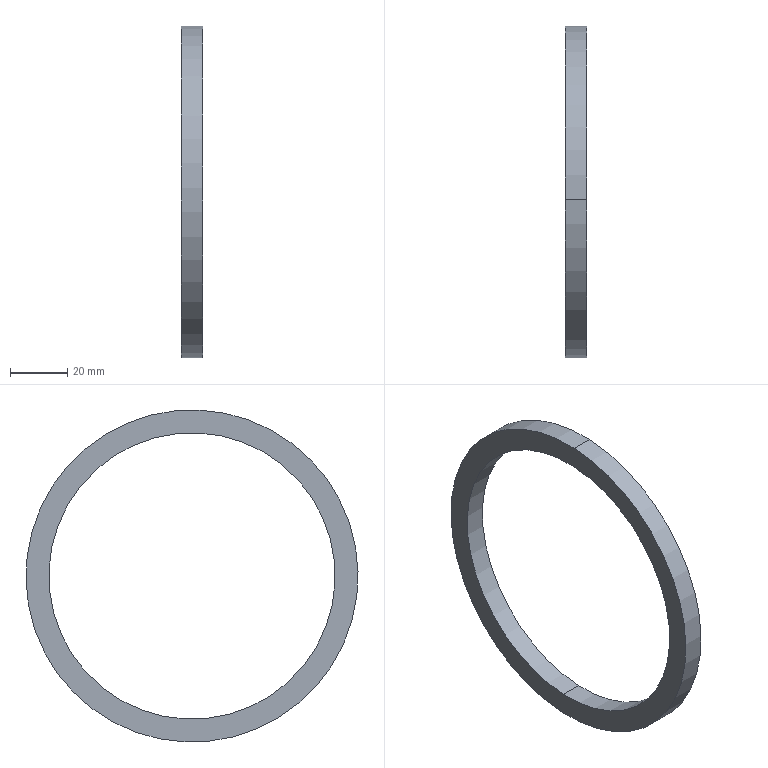Component | SolidWorks | SealRing1-1 | 1 solid | 6 faces | box 7.5 x 116 x 116 mm | volume 20358 mm3 | cylinder 4 | plane 2 | commonest cylinder face diameters 100 x2 116 x2
build123d program:
from build123d import *

# Parameters (mm, degrees)
SKETCH2_R           = 58
SKETCH2_R_2         = 50
BOSS_EXTRUDE1_DEPTH = 7.5


with BuildPart() as part:
    # Sketch2 → Boss-Extrude1 (new body)
    with BuildSketch(Plane(origin=(0, 0, 0), x_dir=(0, 0, -1), z_dir=(1, 0, 0))):
        Circle(SKETCH2_R)
        Circle(SKETCH2_R_2, mode=Mode.SUBTRACT)
    extrude(amount=BOSS_EXTRUDE1_DEPTH)


solid = part.part

# Placed as in the assembly
solid = solid.moved(Location((-138, 0, 0), (0, 0, 0)))
STEP:
#1=COLOUR_RGB('',0.7922,0.8196,0.9333);
#2=FILL_AREA_STYLE_COLOUR('',#1);
#3=FILL_AREA_STYLE('',(#2));
#4=SURFACE_STYLE_FILL_AREA(#3);
#5=SURFACE_SIDE_STYLE('',(#4));
#6=SURFACE_STYLE_USAGE(.BOTH.,#5);
#7=PRESENTATION_STYLE_ASSIGNMENT((#6));
#8=CARTESIAN_POINT('',(-5.138,-0.09506,1.966));
#9=VERTEX_POINT('',#8);
#10=CARTESIAN_POINT('',(-5.138,0.09506,-1.966));
#11=VERTEX_POINT('',#10);
#12=CARTESIAN_POINT('',(-5.138,-0.,0.));
#13=DIRECTION('',(1.,0.,-0.));
#14=DIRECTION('',(-0.,0.04829,-0.9988));
#15=AXIS2_PLACEMENT_3D('',#12,#13,#14);
#16=CIRCLE('',#15,1.969);
#17=EDGE_CURVE('',#9,#11,#16,.T.);
#18=ORIENTED_EDGE('',*,*,#17,.T.);
#19=CARTESIAN_POINT('',(-5.433,0.09506,-1.966));
#20=VERTEX_POINT('',#19);
#21=CARTESIAN_POINT('',(-5.138,0.09506,-1.966));
#22=DIRECTION('',(-1.,-0.,0.));
#23=VECTOR('',#22,39.37);
#24=LINE('',#21,#23);
#25=EDGE_CURVE('',#11,#20,#24,.T.);
#26=ORIENTED_EDGE('',*,*,#25,.T.);
#27=CARTESIAN_POINT('',(-5.433,-0.09506,1.966));
#28=VERTEX_POINT('',#27);
#29=CARTESIAN_POINT('',(-5.433,-0.,0.));
#30=DIRECTION('',(1.,0.,-0.));
#31=DIRECTION('',(-0.,0.04829,-0.9988));
#32=AXIS2_PLACEMENT_3D('',#29,#30,#31);
#33=CIRCLE('',#32,1.969);
#34=EDGE_CURVE('',#28,#20,#33,.T.);
#35=ORIENTED_EDGE('',*,*,#34,.F.);
#36=CARTESIAN_POINT('',(-5.138,-0.09506,1.966));
#37=DIRECTION('',(-1.,-0.,0.));
#38=VECTOR('',#37,39.37);
#39=LINE('',#36,#38);
#40=EDGE_CURVE('',#9,#28,#39,.T.);
#41=ORIENTED_EDGE('',*,*,#40,.F.);
#42=EDGE_LOOP('',(#18,#26,#35,#41));
#43=FACE_OUTER_BOUND('',#42,.T.);
#44=CARTESIAN_POINT('',(-5.138,-0.,0.));
#45=DIRECTION('',(-1.,-0.,0.));
#46=DIRECTION('',(0.,-0.04829,0.9988));
#47=AXIS2_PLACEMENT_3D('',#44,#45,#46);
#48=CYLINDRICAL_SURFACE('',#47,1.969);
#49=ADVANCED_FACE('',(#43),#48,.F.);
#50=CARTESIAN_POINT('',(-5.138,0.1103,-2.281));
#51=VERTEX_POINT('',#50);
#52=CARTESIAN_POINT('',(-5.138,-0.1103,2.281));
#53=VERTEX_POINT('',#52);
#54=CARTESIAN_POINT('',(-5.138,-0.,0.));
#55=DIRECTION('',(1.,0.,-0.));
#56=DIRECTION('',(-0.,0.04829,-0.9988));
#57=AXIS2_PLACEMENT_3D('',#54,#55,#56);
#58=CIRCLE('',#57,2.283);
#59=EDGE_CURVE('',#51,#53,#58,.T.);
#60=ORIENTED_EDGE('',*,*,#59,.F.);
#61=CARTESIAN_POINT('',(-5.433,0.1103,-2.281));
#62=VERTEX_POINT('',#61);
#63=CARTESIAN_POINT('',(-5.138,0.1103,-2.281));
#64=DIRECTION('',(-1.,-0.,0.));
#65=VECTOR('',#64,39.37);
#66=LINE('',#63,#65);
#67=EDGE_CURVE('',#51,#62,#66,.T.);
#68=ORIENTED_EDGE('',*,*,#67,.T.);
#69=CARTESIAN_POINT('',(-5.433,-0.1103,2.281));
#70=VERTEX_POINT('',#69);
#71=CARTESIAN_POINT('',(-5.433,-0.,0.));
#72=DIRECTION('',(1.,0.,-0.));
#73=DIRECTION('',(-0.,0.04829,-0.9988));
#74=AXIS2_PLACEMENT_3D('',#71,#72,#73);
#75=CIRCLE('',#74,2.283);
#76=EDGE_CURVE('',#62,#70,#75,.T.);
#77=ORIENTED_EDGE('',*,*,#76,.T.);
#78=CARTESIAN_POINT('',(-5.138,-0.1103,2.281));
#79=DIRECTION('',(-1.,-0.,0.));
#80=VECTOR('',#79,39.37);
#81=LINE('',#78,#80);
#82=EDGE_CURVE('',#53,#70,#81,.T.);
#83=ORIENTED_EDGE('',*,*,#82,.F.);
#84=EDGE_LOOP('',(#60,#68,#77,#83));
#85=FACE_OUTER_BOUND('',#84,.T.);
#86=CARTESIAN_POINT('',(-5.138,-0.,0.));
#87=DIRECTION('',(-1.,-0.,0.));
#88=DIRECTION('',(0.,-0.04829,0.9988));
#89=AXIS2_PLACEMENT_3D('',#86,#87,#88);
#90=CYLINDRICAL_SURFACE('',#89,2.283);
#91=ADVANCED_FACE('',(#85),#90,.T.);
#92=CARTESIAN_POINT('',(-5.138,-0.,0.));
#93=DIRECTION('',(1.,0.,-0.));
#94=DIRECTION('',(-0.,0.04829,-0.9988));
#95=AXIS2_PLACEMENT_3D('',#92,#93,#94);
#96=CIRCLE('',#95,2.283);
#97=EDGE_CURVE('',#53,#51,#96,.T.);
#98=ORIENTED_EDGE('',*,*,#97,.T.);
#99=ORIENTED_EDGE('',*,*,#59,.T.);
#100=EDGE_LOOP('',(#98,#99));
#101=FACE_OUTER_BOUND('',#100,.T.);
#102=ORIENTED_EDGE('',*,*,#17,.F.);
#103=CARTESIAN_POINT('',(-5.138,-0.,0.));
#104=DIRECTION('',(1.,0.,-0.));
#105=DIRECTION('',(-0.,0.04829,-0.9988));
#106=AXIS2_PLACEMENT_3D('',#103,#104,#105);
#107=CIRCLE('',#106,1.969);
#108=EDGE_CURVE('',#11,#9,#107,.T.);
#109=ORIENTED_EDGE('',*,*,#108,.F.);
#110=EDGE_LOOP('',(#102,#109));
#111=FACE_BOUND('',#110,.T.);
#112=CARTESIAN_POINT('',(-5.138,-0.,0.));
#113=DIRECTION('',(1.,0.,-0.));
#114=DIRECTION('',(-0.,0.04829,-0.9988));
#115=AXIS2_PLACEMENT_3D('',#112,#113,#114);
#116=PLANE('',#115);
#117=ADVANCED_FACE('',(#101,#111),#116,.T.);
#118=CARTESIAN_POINT('',(-5.433,-0.,0.));
#119=DIRECTION('',(1.,0.,-0.));
#120=DIRECTION('',(-0.,0.04829,-0.9988));
#121=AXIS2_PLACEMENT_3D('',#118,#119,#120);
#122=CIRCLE('',#121,2.283);
#123=EDGE_CURVE('',#70,#62,#122,.T.);
#124=ORIENTED_EDGE('',*,*,#123,.F.);
#125=ORIENTED_EDGE('',*,*,#76,.F.);
#126=EDGE_LOOP('',(#124,#125));
#127=FACE_OUTER_BOUND('',#126,.T.);
#128=ORIENTED_EDGE('',*,*,#34,.T.);
#129=CARTESIAN_POINT('',(-5.433,-0.,0.));
#130=DIRECTION('',(1.,0.,-0.));
#131=DIRECTION('',(-0.,0.04829,-0.9988));
#132=AXIS2_PLACEMENT_3D('',#129,#130,#131);
#133=CIRCLE('',#132,1.969);
#134=EDGE_CURVE('',#20,#28,#133,.T.);
#135=ORIENTED_EDGE('',*,*,#134,.T.);
#136=EDGE_LOOP('',(#128,#135));
#137=FACE_BOUND('',#136,.T.);
#138=CARTESIAN_POINT('',(-5.433,-0.,0.));
#139=DIRECTION('',(1.,0.,-0.));
#140=DIRECTION('',(-0.,0.04829,-0.9988));
#141=AXIS2_PLACEMENT_3D('',#138,#139,#140);
#142=PLANE('',#141);
#143=ADVANCED_FACE('',(#127,#137),#142,.F.);
#144=ORIENTED_EDGE('',*,*,#67,.F.);
#145=ORIENTED_EDGE('',*,*,#97,.F.);
#146=ORIENTED_EDGE('',*,*,#82,.T.);
#147=ORIENTED_EDGE('',*,*,#123,.T.);
#148=EDGE_LOOP('',(#144,#145,#146,#147));
#149=FACE_OUTER_BOUND('',#148,.T.);
#150=CARTESIAN_POINT('',(-5.138,-0.,0.));
#151=DIRECTION('',(-1.,-0.,0.));
#152=DIRECTION('',(0.,-0.04829,0.9988));
#153=AXIS2_PLACEMENT_3D('',#150,#151,#152);
#154=CYLINDRICAL_SURFACE('',#153,2.283);
#155=ADVANCED_FACE('',(#149),#154,.T.);
#156=ORIENTED_EDGE('',*,*,#25,.F.);
#157=ORIENTED_EDGE('',*,*,#108,.T.);
#158=ORIENTED_EDGE('',*,*,#40,.T.);
#159=ORIENTED_EDGE('',*,*,#134,.F.);
#160=EDGE_LOOP('',(#156,#157,#158,#159));
#161=FACE_OUTER_BOUND('',#160,.T.);
#162=CARTESIAN_POINT('',(-5.138,-0.,0.));
#163=DIRECTION('',(-1.,-0.,0.));
#164=DIRECTION('',(0.,-0.04829,0.9988));
#165=AXIS2_PLACEMENT_3D('',#162,#163,#164);
#166=CYLINDRICAL_SURFACE('',#165,1.969);
#167=ADVANCED_FACE('',(#161),#166,.F.);
#168=CLOSED_SHELL('',(#49,#91,#117,#143,#155,#167));
#169=MANIFOLD_SOLID_BREP('',#168);
#170=STYLED_ITEM('',(#7),#169);
#171=(LENGTH_UNIT()NAMED_UNIT(*)SI_UNIT($,.METRE.));
#172=LENGTH_MEASURE_WITH_UNIT(LENGTH_MEASURE(0.0254),#171);
#173=DIMENSIONAL_EXPONENTS(1.,0.,0.,0.,0.,0.,0.);
#174=(CONVERSION_BASED_UNIT('',#172)LENGTH_UNIT()NAMED_UNIT(#173));
#175=UNCERTAINTY_MEASURE_WITH_UNIT(LENGTH_MEASURE(0.00001),#174,'','');
#176=(NAMED_UNIT(*)PLANE_ANGLE_UNIT()SI_UNIT($,.RADIAN.));
#177=(NAMED_UNIT(*)SI_UNIT($,.STERADIAN.)SOLID_ANGLE_UNIT());
#178=(GEOMETRIC_REPRESENTATION_CONTEXT(3)GLOBAL_UNCERTAINTY_ASSIGNED_CONTEXT((#175))GLOBAL_UNIT_ASSIGNED_CONTEXT((#174,#176,#177))REPRESENTATION_CONTEXT('',''));
#179=MECHANICAL_DESIGN_GEOMETRIC_PRESENTATION_REPRESENTATION('',(#170),#178);
#180=CARTESIAN_POINT('',(0.,0.,0.));
#181=DIRECTION('',(0.,0.,1.));
#182=DIRECTION('',(1.,0.,0.));
#183=AXIS2_PLACEMENT_3D('',#180,#181,#182);
#184=(LENGTH_UNIT()NAMED_UNIT(*)SI_UNIT($,.METRE.));
#185=LENGTH_MEASURE_WITH_UNIT(LENGTH_MEASURE(0.0254),#184);
#186=DIMENSIONAL_EXPONENTS(1.,0.,0.,0.,0.,0.,0.);
#187=(CONVERSION_BASED_UNIT('',#185)LENGTH_UNIT()NAMED_UNIT(#186));
#188=UNCERTAINTY_MEASURE_WITH_UNIT(LENGTH_MEASURE(0.00001),#187,'','');
#189=(NAMED_UNIT(*)PLANE_ANGLE_UNIT()SI_UNIT($,.RADIAN.));
#190=(NAMED_UNIT(*)SI_UNIT($,.STERADIAN.)SOLID_ANGLE_UNIT());
#191=(GEOMETRIC_REPRESENTATION_CONTEXT(3)GLOBAL_UNCERTAINTY_ASSIGNED_CONTEXT((#188))GLOBAL_UNIT_ASSIGNED_CONTEXT((#187,#189,#190))REPRESENTATION_CONTEXT('',''));
#192=ADVANCED_BREP_SHAPE_REPRESENTATION('',(#169,#183),#191);
#193=PRESENTATION_LAYER_ASSIGNMENT('','',(#170));